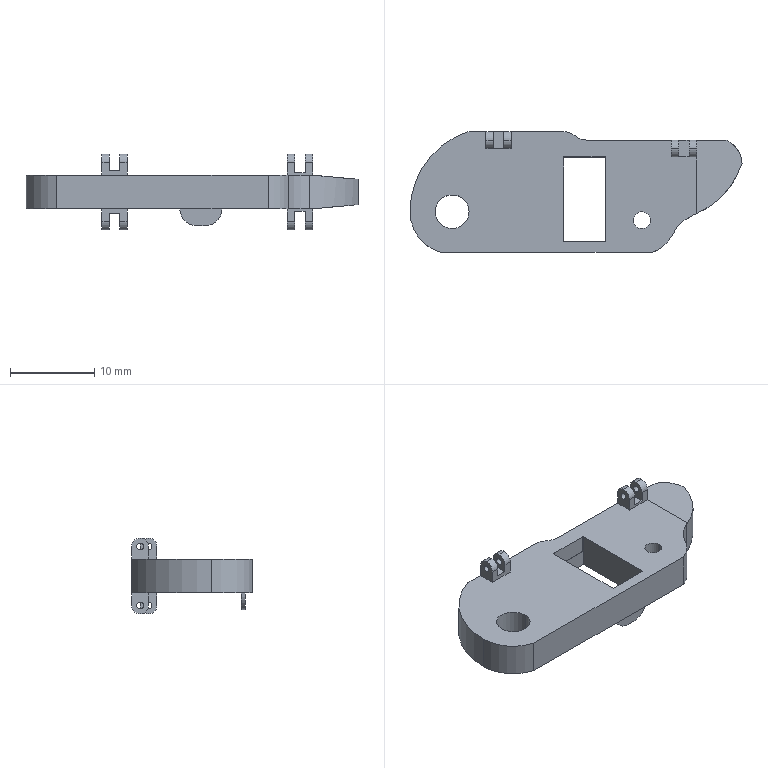Component | SolidWorks | Fuselage-1 | 1 solid | 87 faces | volume 1647 mm3 | cylinder 46 | plane 41 | commonest cylinder face diameters 2 x18 0.8 x16 4 x6 10 x2 20 x2 8 x1 6 x1